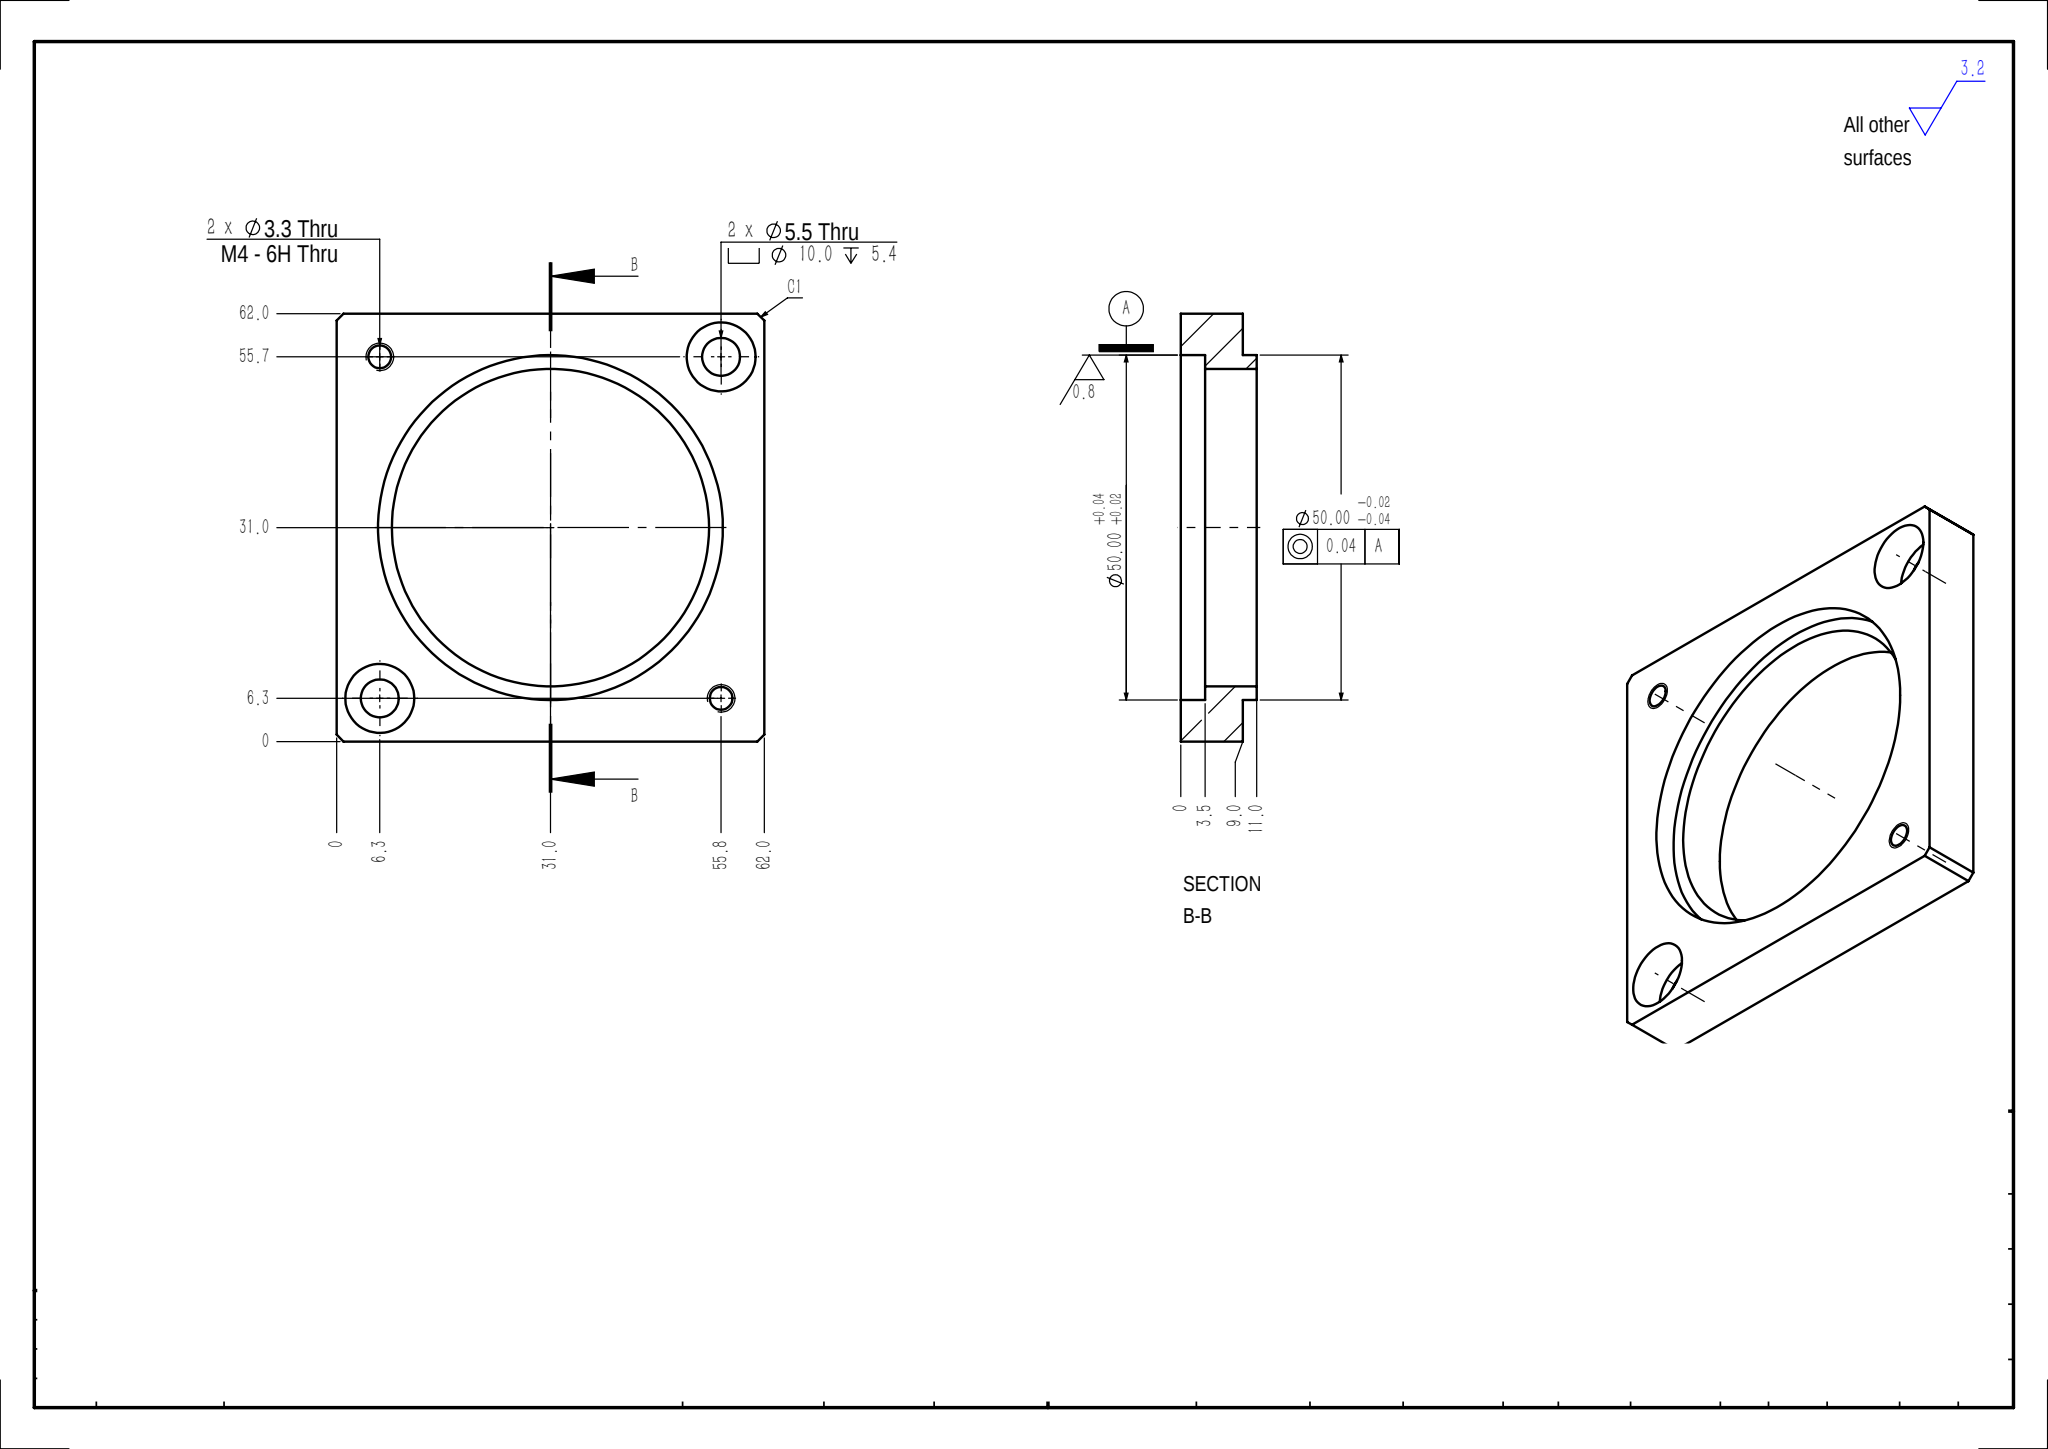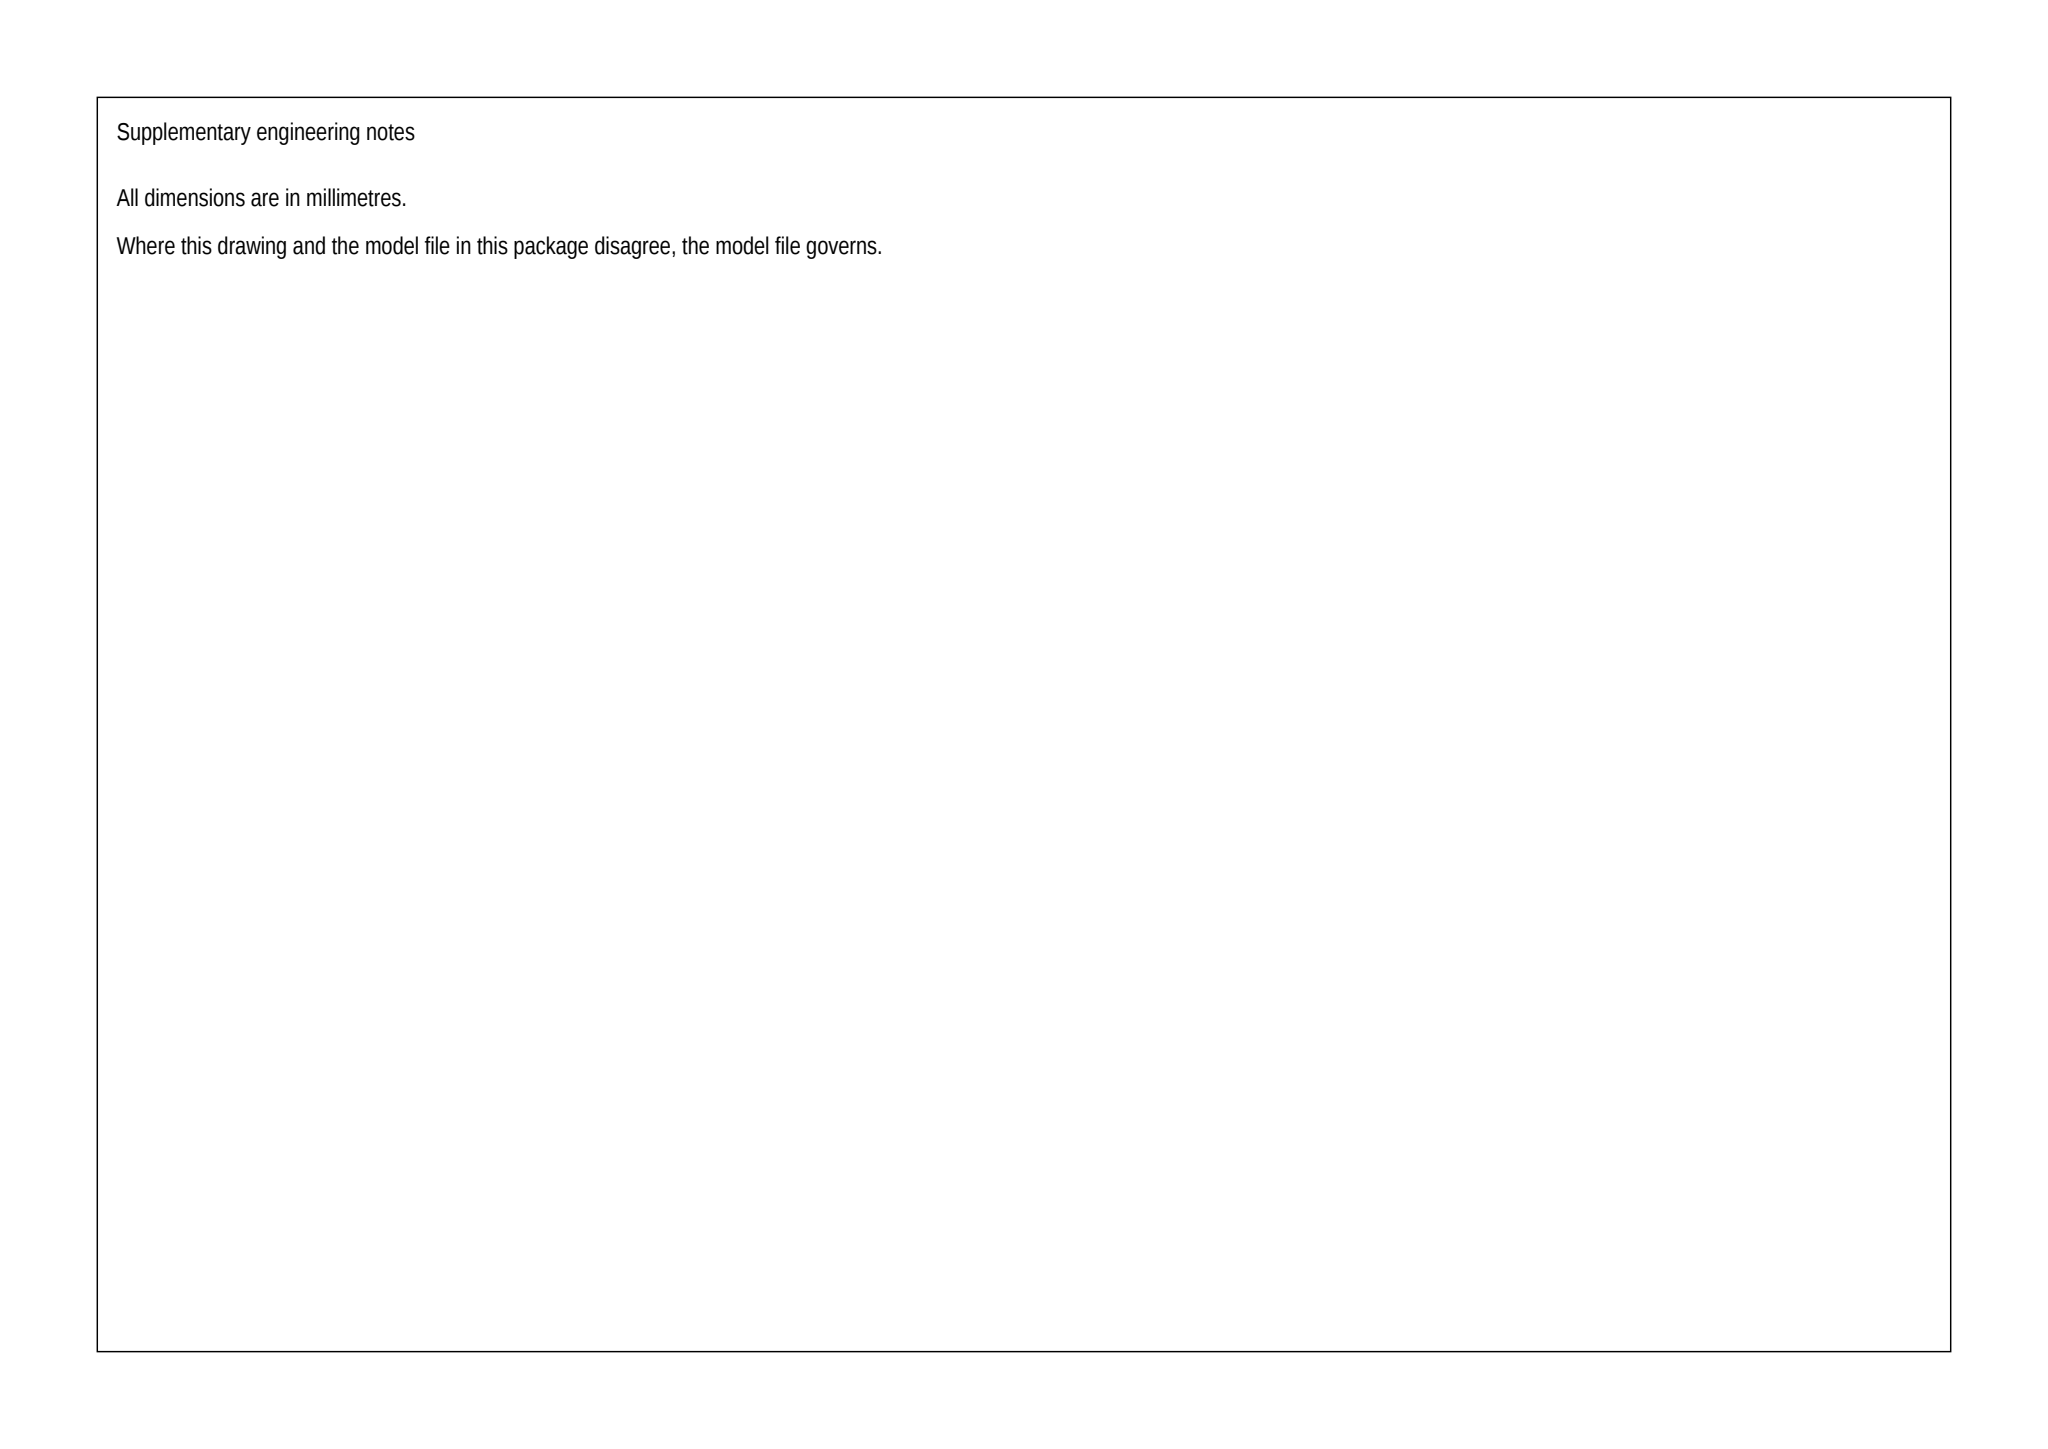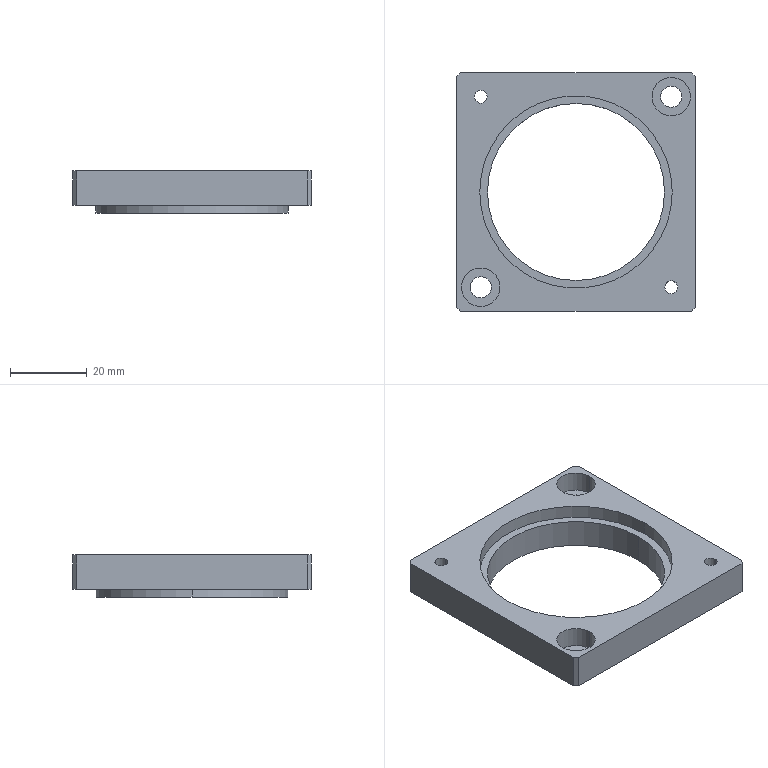Part | SolidWorks | mm | 1 solid | 32 faces | box 62 x 62 x 11 mm | volume 17995 mm3 | cylinder 18 | plane 14 | commonest cylinder face diameters 10 x4 5.5 x4 3.3 x4 50 x4 46 x2
build123d program:
from build123d import *

# Parameters (mm, degrees)
SKETCH1_W                                       = 62
SKETCH1_H                                       = 62
BOSS_EXTRUDE1_DEPTH                             = 5.5
SKETCH2_W                                       = 62
SKETCH2_H                                       = 62
SKETCH2_R                                       = 25
CUT_EXTRUDE1_DEPTH                              = 2
SKETCH3_R                                       = 23
CUT_EXTRUDE2_DEPTH                              = 46.2
CUT_EXTRUDE3_START                              = -3.5
SKETCH4_R                                       = 25
CUT_EXTRUDE3_DEPTH                              = 3.5
M4_TAPPED_HOLE1_D                               = 3.3
M5_HEX_SOCKET_HEAD_CAP_SCREW_CBORE1_D           = 5.5
M5_HEX_SOCKET_HEAD_CAP_SCREW_CBORE1_CBORE_D     = 10
M5_HEX_SOCKET_HEAD_CAP_SCREW_CBORE1_CBORE_DEPTH = 5.4
CHAMFER1_SIZE                                   = 1


with BuildPart() as part:
    # Sketch1 → Boss-Extrude1 (new, symmetric)
    with BuildSketch(Plane.XY):
        Rectangle(SKETCH1_W, SKETCH1_H)
    extrude(amount=BOSS_EXTRUDE1_DEPTH, both=True)

    # Sketch2 → Cut-Extrude1 (cut)
    with BuildSketch(Plane(origin=(0, 0, -5.5), x_dir=(-1, 0, 0), z_dir=(0, 0, -1))):
        Rectangle(SKETCH2_W, SKETCH2_H)
        Circle(SKETCH2_R, mode=Mode.SUBTRACT)
    extrude(amount=-CUT_EXTRUDE1_DEPTH, mode=Mode.SUBTRACT)

    # Sketch3 → Cut-Extrude2 (cut, through all)
    with BuildSketch(Plane(origin=(0, 0, -5.5), x_dir=(-1, 0, 0), z_dir=(0, 0, -1))):
        Circle(SKETCH3_R)
    extrude(amount=-CUT_EXTRUDE2_DEPTH, mode=Mode.SUBTRACT)

    # Sketch4 → Cut-Extrude3 (cut)
    with BuildSketch(Plane.XY.offset(5.5).offset(CUT_EXTRUDE3_START)):
        with Locations(Location((0, 0, 0), (0, 0, 180))):
            Circle(SKETCH4_R)
    extrude(amount=CUT_EXTRUDE3_DEPTH, mode=Mode.SUBTRACT)

    # M4 Tapped Hole1 (through all)
    with Locations(Plane.XY.offset(5.5)):
        with Locations((24.75, -24.747), (-24.75, 24.747)):
            Hole(M4_TAPPED_HOLE1_D / 2)

    # M5 Hex Socket Head Cap Screw CBORE1 (through all)
    with Locations(Plane.XY.offset(5.5)):
        with Locations((24.75, 24.747), (-24.75, -24.747)):
            CounterBoreHole(M5_HEX_SOCKET_HEAD_CAP_SCREW_CBORE1_D / 2, M5_HEX_SOCKET_HEAD_CAP_SCREW_CBORE1_CBORE_D / 2, M5_HEX_SOCKET_HEAD_CAP_SCREW_CBORE1_CBORE_DEPTH)

    # Chamfer1
    chamfer1_edges = [part.edges().sort_by_distance(p)[0] for p in [
        (31, -31, 1),
        (-31, -31, 1),
        (-31, 31, 1),
        (31, 31, 1),
    ]]
    chamfer(chamfer1_edges, length=CHAMFER1_SIZE)


solid = part.part